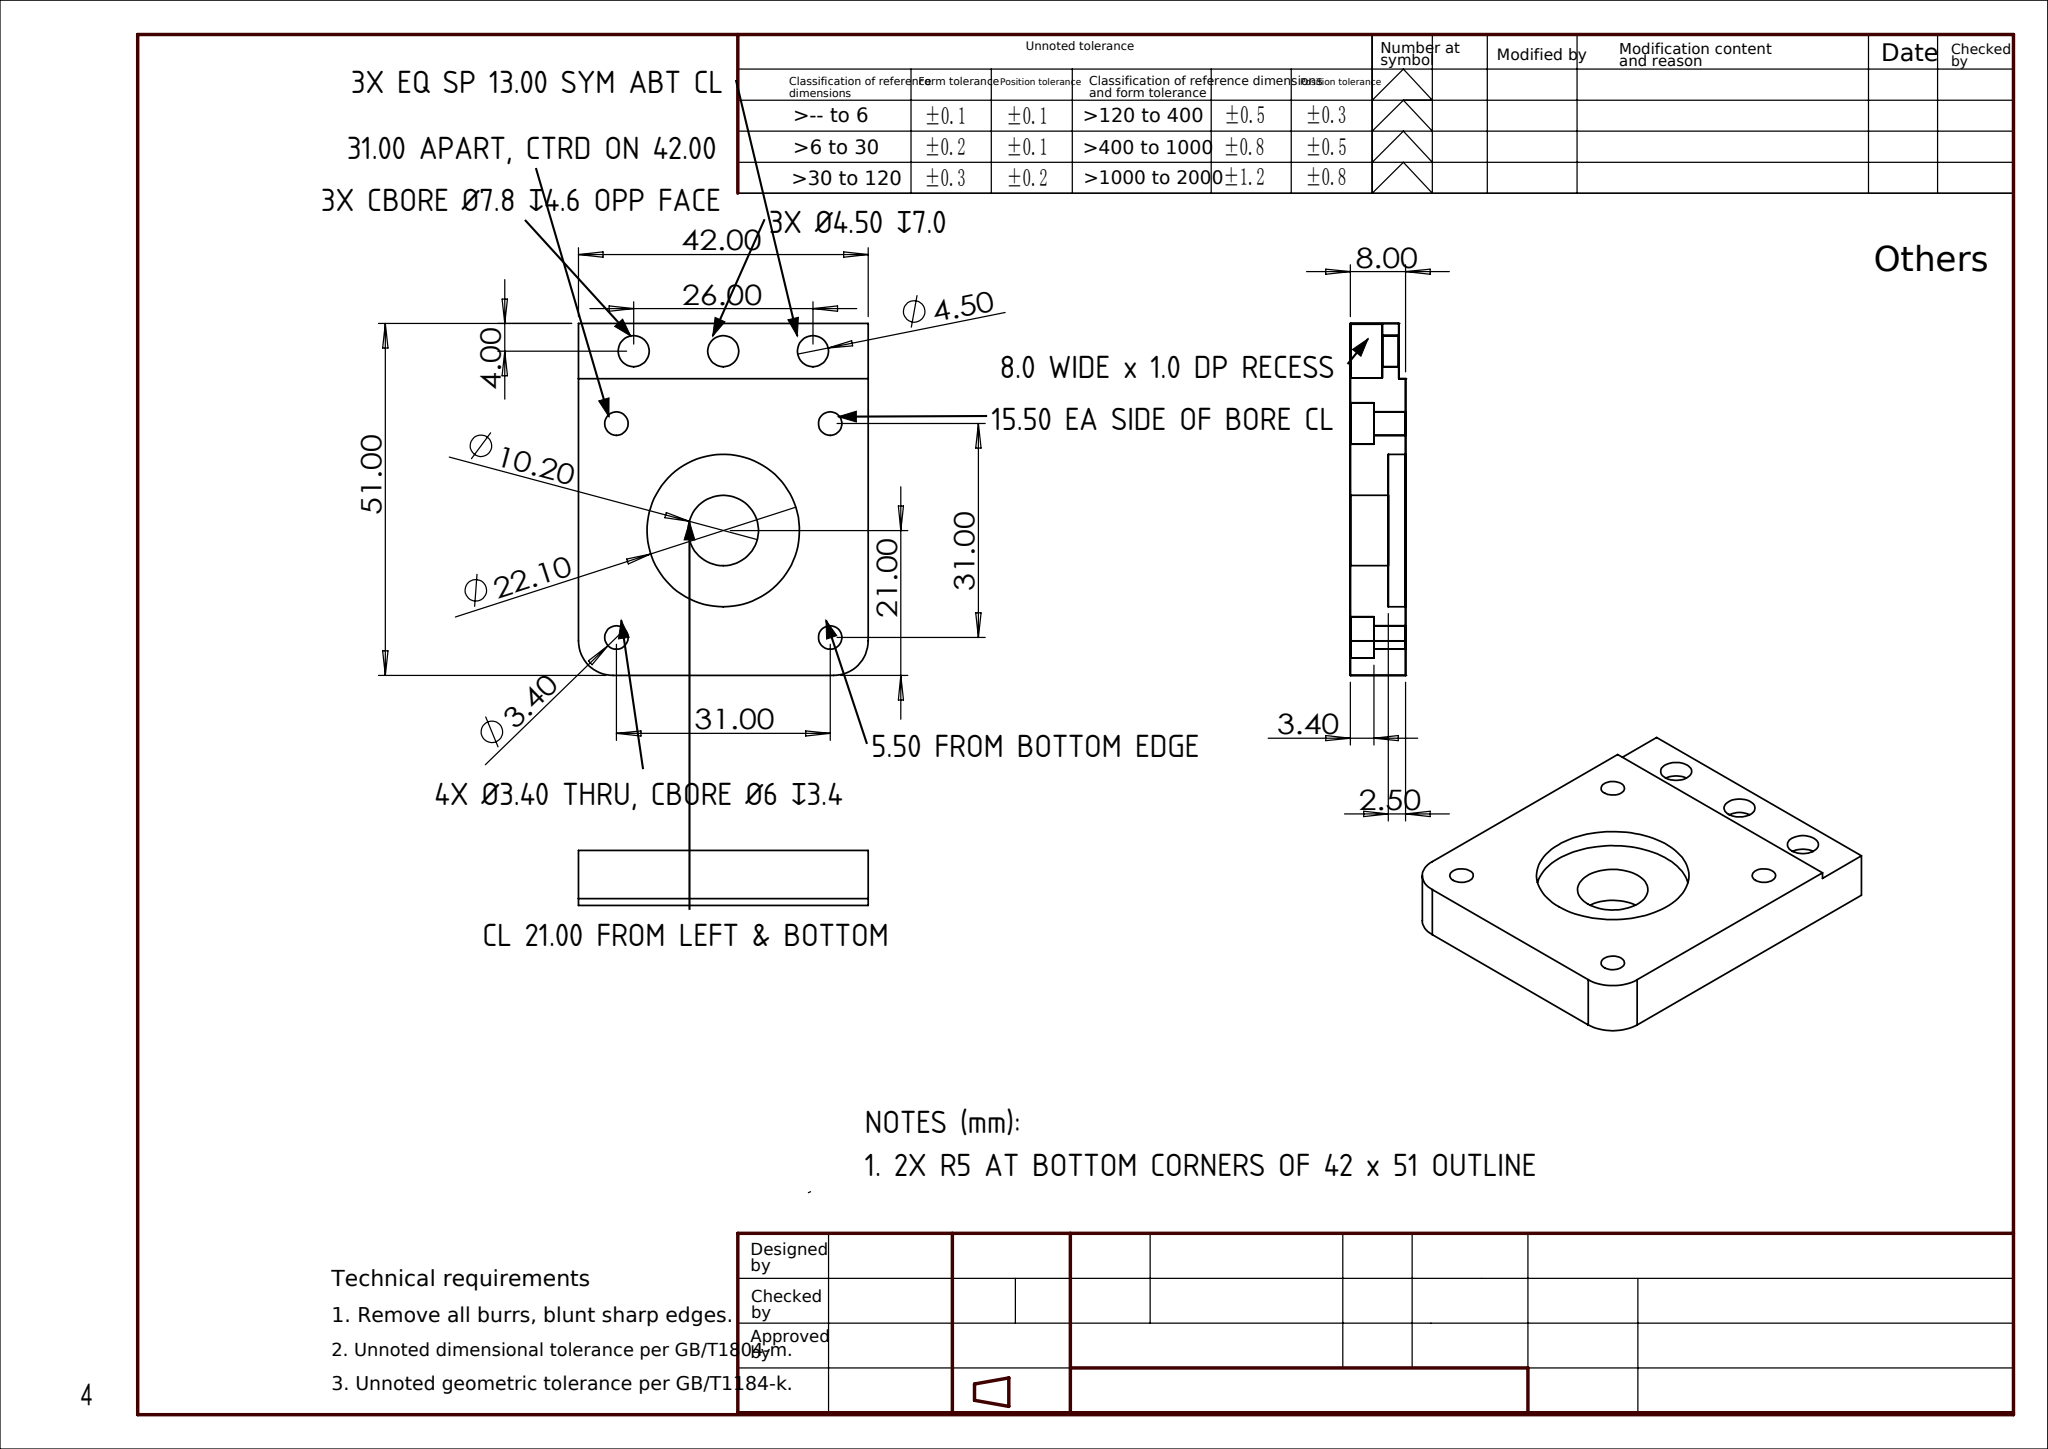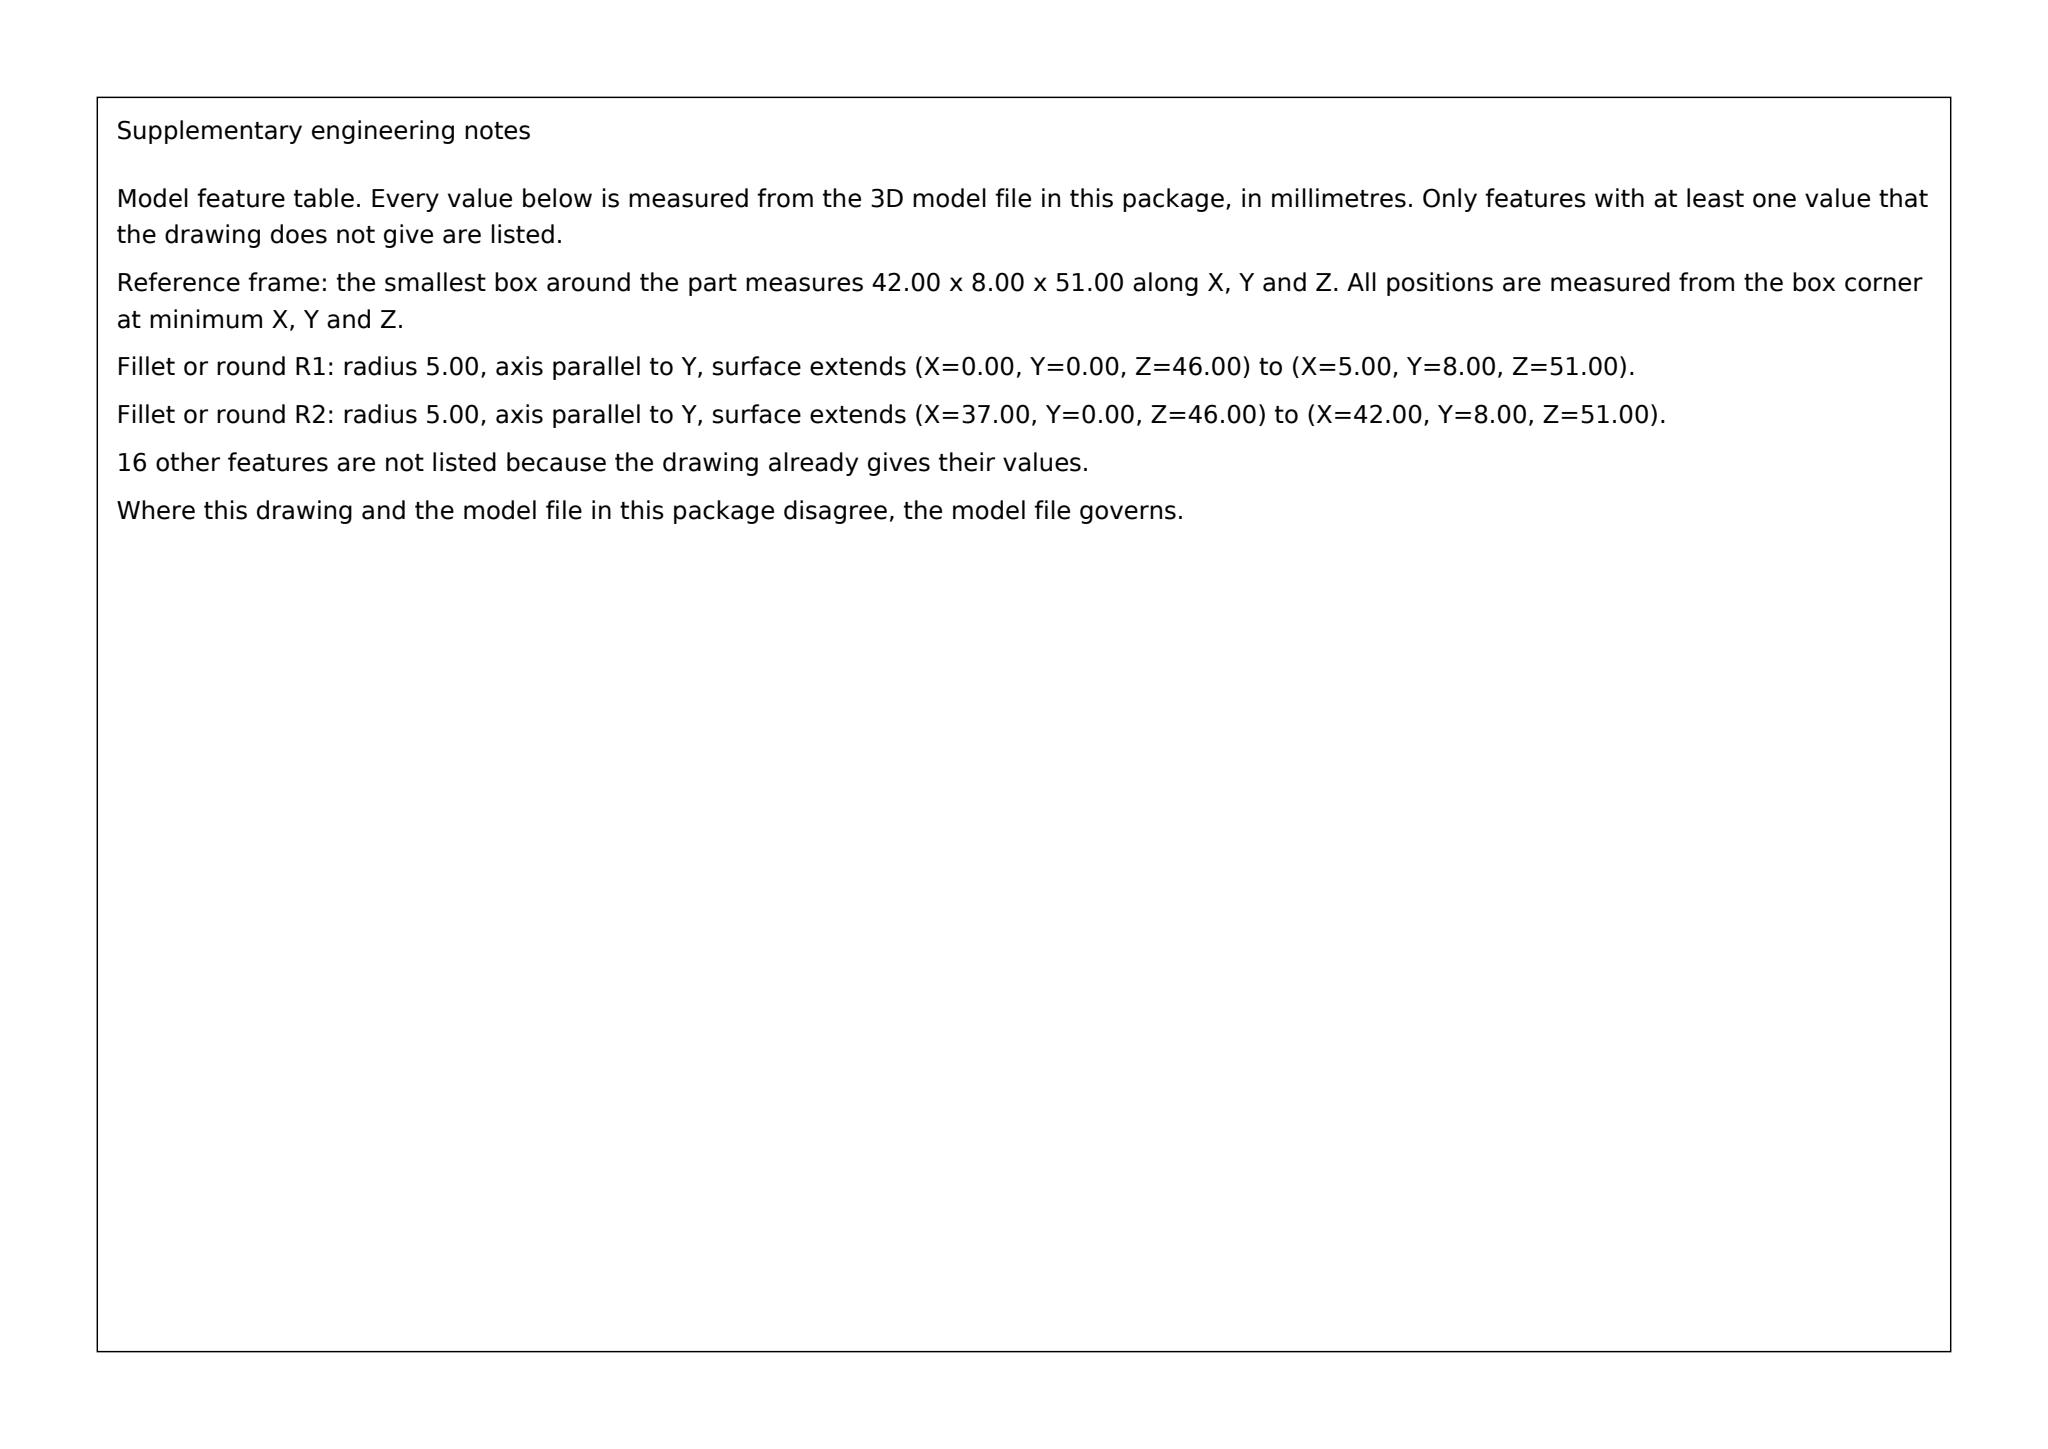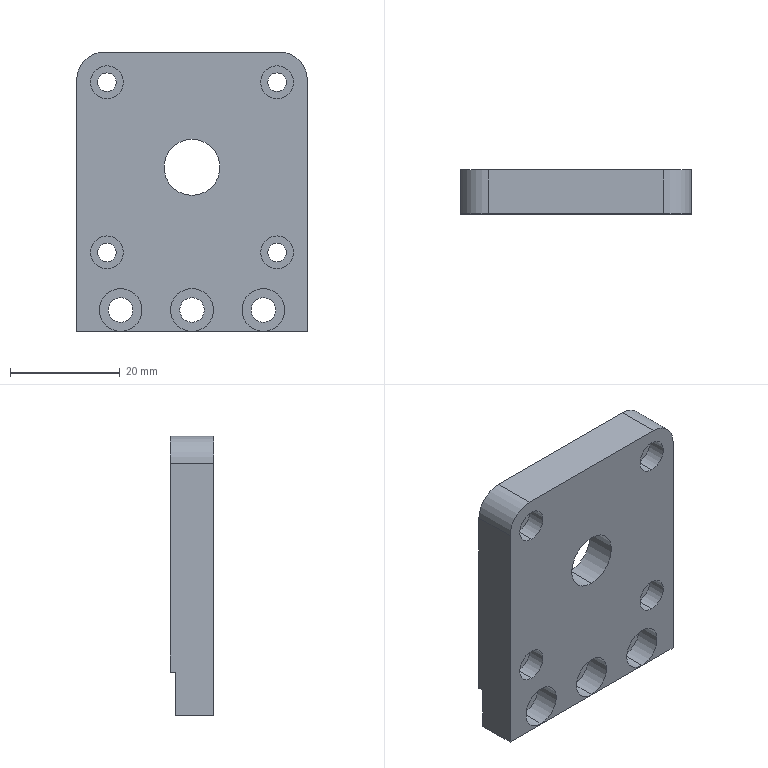Part | SolidWorks | mm | 1 solid | 50 faces | box 42 x 8 x 51 mm | volume 13980 mm3 | cylinder 34 | plane 16 | commonest cylinder face diameters 6 x8 3.4 x8 7.8 x6 4.5 x6 22.1 x2 10.2 x2 10 x2
Drawing notes:
4X Ø3.40 THRU, C'BORE Ø6.0 DP 3.4 FROM OPP (C'BORE) FACE | from the solid: Ø6.0 y-cyl L=3.4 at (5.5/36.5, 14.5/45.5) over Ø3.4 L=4.6; y-plane 3.4 x4
3X Ø4.50: C'BORE Ø7.8 DP 4.6 FROM OPP (C'BORE) FACE | from the solid: Ø7.8 y-cyl L=4.6 at x=8,21,34 z=4.0; y-plane 4.6 count 3
3X Ø4.50 DP 7.0 FROM C'BORE FACE, EXITS IN RECESSED BAND | from the solid: Ø4.5 y-cyl L=2.4 after 4.6 c'bore = ends at y=7.0; band face y=7.0, not 8.0
2X R5 AT BOTTOM CORNERS OF 42 x 51 OUTLINE | from the solid: Ø10.0 y-cyl L=8.0 (full thk) at (5.0,46.0) and (37.0,46.0) = R5, 5 from edges
TOP BAND 8.0 WIDE x 1.0 DEEP RECESS ON Ø22.10 FACE | from the solid: y-plane 7.0 (1.0 below face y=8.0); z-plane 8.0 step wall; holes at z=4.0 in band
4X Ø3.40 ROWS SYM ABT Ø10.20 BORE CL: 15.50 EA SIDE (31.00 APART) | from the solid: Ø3.4 holes at z=14.5 & 45.5; Ø10.2 bore at z=30.0 -> 15.5 each side
4X Ø3.40 C'BORE PATTERN CTRD ON 42.00 WIDTH: 31.00 APART (15.50 EA) | from the solid: Ø3.4 holes at x=5.5 & 36.5 in 42.0 wide bbox -> sym about x=21.0
LOWER Ø3.40 ROW 5.50 FROM BOTTOM EDGE OF 51.00 OUTLINE | from the solid: z=45.5 in 51.0 tall bbox; bottom edge datum used by 21.00 dim
3X Ø4.50 EQ SP 13.00 APART, PATTERN SYM ABOUT 42.00 WIDTH CL: HOLE CENTRES AT 8.00, 21.00 AND 34.00 FROM LEFT EDGE | from the solid: cylinders dia 4.5 axis y at x=8.0, 21.0, 34.0 (z=4.0); bbox_xyz x=42.0 so centre hole on 21.00 CL, 13.00 spacing
Ø10.20 CENTRAL BORE THRU, 5.50 DEEP BELOW Ø22.10 x 2.50 DP C'BORE (8.00 TOTAL = PLATE THICKNESS), ON BORE CL 21.00 FROM LEFT EDGE AND 21.00 FROM BOTTOM EDGE | from the solid: cylinder [10.2,y,[21.0,null,30.0],5.5] + cylinder [22.1,y,[21.0,null,30.0],2.5]; bbox y=8.0 (2.5+5.5=8.0 thru)
build123d program:
from build123d import *

# Parameters (mm, degrees)
SKETCH1_W                                         = 42
SKETCH1_H                                         = 51
BOSS_EXTRUDE1_DEPTH                               = 8
SKETCH4_W                                         = 42
SKETCH4_H                                         = 8
CUT_EXTRUDE3_DEPTH                                = 1
HOLE_SIZE_ACCORDING_TO_HEXAGON_SOCKET_D           = 4.5
HOLE_SIZE_ACCORDING_TO_HEXAGON_SOCKET_CBORE_D     = 7.8
HOLE_SIZE_ACCORDING_TO_HEXAGON_SOCKET_CBORE_DEPTH = 4.6
SKETCH7_R                                         = 5.1
CUT_EXTRUDE4_DEPTH                                = 10
SKETCH8_R                                         = 11.05
CUT_EXTRUDE5_DEPTH                                = 2.5
FILLET1_R                                         = 5
HOLE_SIZE_ACCORDING_TO_HEXAGON_SO_2_D             = 3.4
HOLE_SIZE_ACCORDING_TO_HEXAGON_SO_2_DEPTH         = 23
HOLE_SIZE_ACCORDING_TO_HEXAGON_SO_2_CBORE_D       = 6
HOLE_SIZE_ACCORDING_TO_HEXAGON_SO_2_CBORE_DEPTH   = 3.4
HOLE_SIZE_ACCORDING_TO_HEXAGON_SO_2_TIP           = 1.021


with BuildPart() as part:
    # Sketch1 → Boss-Extrude1 (new body)
    with BuildSketch(Plane(origin=(0, 0, 0), x_dir=(1, 0, 0), z_dir=(0, 1, 0))):
        Rectangle(SKETCH1_W, SKETCH1_H)
    extrude(amount=BOSS_EXTRUDE1_DEPTH)

    # Sketch4 → Cut-Extrude3 (cut)
    with BuildSketch(Plane(origin=(0, 8, 0), x_dir=(1, 0, 0), z_dir=(0, 1, 0))):
        with Locations((0, 21.5)):
            Rectangle(SKETCH4_W, SKETCH4_H)
    extrude(amount=-CUT_EXTRUDE3_DEPTH, mode=Mode.SUBTRACT)

    # Hole Size _ according to_ Hexagon Socket (through all)
    with Locations(Plane(origin=(0, 0, 0), x_dir=(-1, 0, 0), z_dir=(0, -1, 0))):
        with Locations((-13, 21.5), (0, 21.5), (13, 21.5)):
            CounterBoreHole(HOLE_SIZE_ACCORDING_TO_HEXAGON_SOCKET_D / 2, HOLE_SIZE_ACCORDING_TO_HEXAGON_SOCKET_CBORE_D / 2, HOLE_SIZE_ACCORDING_TO_HEXAGON_SOCKET_CBORE_DEPTH)

    # Sketch7 → Cut-Extrude4 (cut)
    with BuildSketch(Plane.XZ):
        with Locations(Location((0, 4.5, 0), (0, 0, 270))):
            Circle(SKETCH7_R)
    extrude(amount=-CUT_EXTRUDE4_DEPTH, mode=Mode.SUBTRACT)

    # Sketch8 → Cut-Extrude5 (cut)
    with BuildSketch(Plane(origin=(0, 8, 0), x_dir=(1, 0, 0), z_dir=(0, 1, 0))):
        with Locations(Location((0, -4.5, 0), (0, 0, 270))):
            Circle(SKETCH8_R)
    extrude(amount=-CUT_EXTRUDE5_DEPTH, mode=Mode.SUBTRACT)

    # Fillet1
    fillet1_edges = [part.edges().sort_by_distance(p)[0] for p in [
        (21, 4, 25.5),
        (-21, 4, 25.5),
    ]]
    fillet(fillet1_edges, radius=FILLET1_R)

    # Hole Size _ according to_ Hexagon So 2
    with Locations(Plane(origin=(0, 0, 0), x_dir=(-1, 0, 0), z_dir=(0, -1, 0))):
        with Locations((15.5, 11), (-15.5, 11), (-15.5, -20), (15.5, -20)):
            CounterBoreHole(HOLE_SIZE_ACCORDING_TO_HEXAGON_SO_2_D / 2, HOLE_SIZE_ACCORDING_TO_HEXAGON_SO_2_CBORE_D / 2, HOLE_SIZE_ACCORDING_TO_HEXAGON_SO_2_CBORE_DEPTH, depth=HOLE_SIZE_ACCORDING_TO_HEXAGON_SO_2_DEPTH)
            with Locations((0, 0, -(HOLE_SIZE_ACCORDING_TO_HEXAGON_SO_2_DEPTH + HOLE_SIZE_ACCORDING_TO_HEXAGON_SO_2_TIP / 2))):  # 118° drill point
                Cone(0, HOLE_SIZE_ACCORDING_TO_HEXAGON_SO_2_D / 2, HOLE_SIZE_ACCORDING_TO_HEXAGON_SO_2_TIP, mode=Mode.SUBTRACT)


solid = part.part